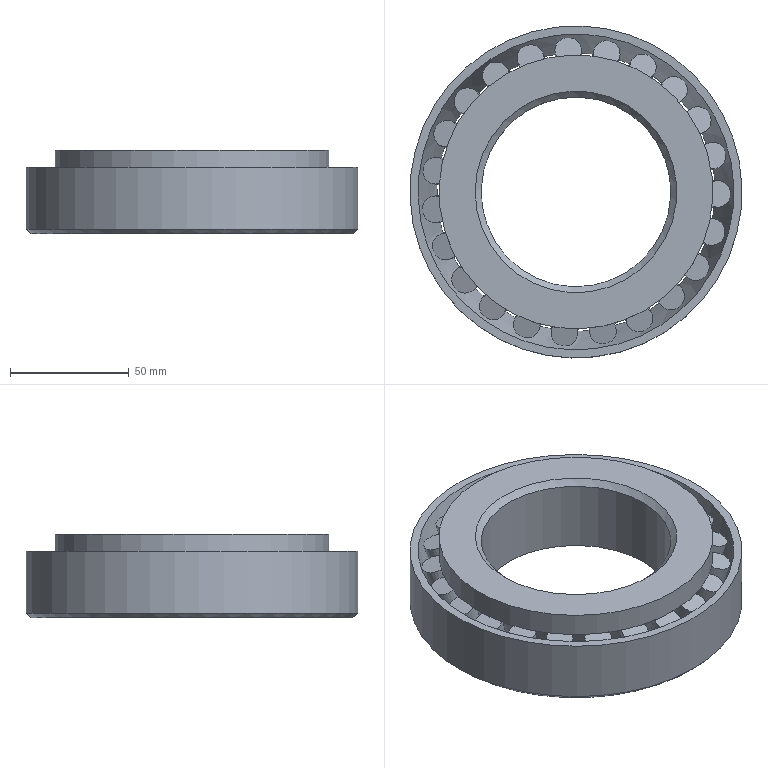Component | NX | CA6140-ZHUZHOU-7516E-32216 | 25 solids | 81 faces | volume 254969 mm3 | plane 50 | cylinder 26 | cone 5 | commonest cylinder face diameters 11.267 x23 115.466 x1 80 x1 140 x1